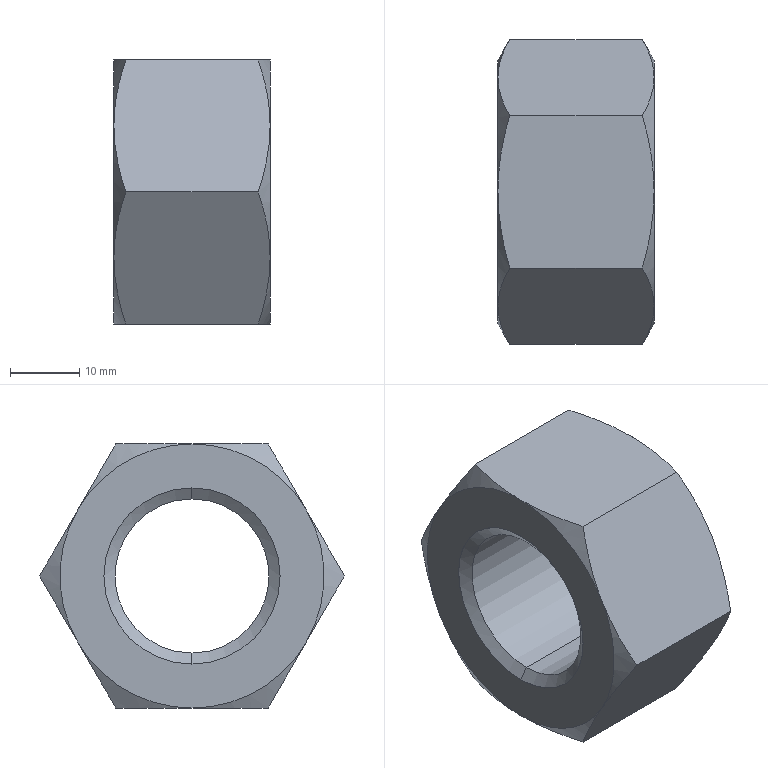Component | SolidWorks | hex thin nut chamfered gradeab_iso-1 | 1 solid | 28 faces | box 22.53 x 43.99 x 38.1 mm | volume 19330 mm3 | cone 16 | plane 8 | cylinder 4 | commonest cylinder face diameters 25.4 x2 22.225 x2
STEP:
#1=CARTESIAN_POINT('',(1.476,2.362,-4.831));
#2=VERTEX_POINT('',#1);
#3=CARTESIAN_POINT('',(1.476,2.362,-3.831));
#4=VERTEX_POINT('',#3);
#5=CARTESIAN_POINT('',(1.476,2.362,-4.331));
#6=DIRECTION('',(-1.,0.,0.));
#7=DIRECTION('',(0.,0.,-1.));
#8=AXIS2_PLACEMENT_3D('',#5,#6,#7);
#9=CIRCLE('',#8,0.5);
#10=EDGE_CURVE('',#2,#4,#9,.T.);
#11=ORIENTED_EDGE('',*,*,#10,.T.);
#12=CARTESIAN_POINT('',(1.477,2.362,-3.831));
#13=VERTEX_POINT('',#12);
#14=CARTESIAN_POINT('',(1.378,2.362,-3.831));
#15=DIRECTION('',(1.,0.,0.));
#16=VECTOR('',#15,39.37);
#17=LINE('',#14,#16);
#18=EDGE_CURVE('',#4,#13,#17,.T.);
#19=ORIENTED_EDGE('',*,*,#18,.T.);
#20=CARTESIAN_POINT('',(1.477,2.362,-4.831));
#21=VERTEX_POINT('',#20);
#22=CARTESIAN_POINT('',(1.477,2.362,-4.331));
#23=DIRECTION('',(1.,0.,0.));
#24=DIRECTION('',(0.,0.,-1.));
#25=AXIS2_PLACEMENT_3D('',#22,#23,#24);
#26=CIRCLE('',#25,0.5);
#27=EDGE_CURVE('',#13,#21,#26,.T.);
#28=ORIENTED_EDGE('',*,*,#27,.T.);
#29=CARTESIAN_POINT('',(1.378,2.362,-4.831));
#30=DIRECTION('',(1.,0.,0.));
#31=VECTOR('',#30,39.37);
#32=LINE('',#29,#31);
#33=EDGE_CURVE('',#2,#21,#32,.T.);
#34=ORIENTED_EDGE('',*,*,#33,.F.);
#35=EDGE_LOOP('',(#11,#19,#28,#34));
#36=FACE_OUTER_BOUND('',#35,.T.);
#37=CARTESIAN_POINT('',(1.378,2.362,-4.331));
#38=DIRECTION('',(1.,0.,0.));
#39=DIRECTION('',(0.,0.,-1.));
#40=AXIS2_PLACEMENT_3D('',#37,#38,#39);
#41=CYLINDRICAL_SURFACE('',#40,0.5);
#42=ADVANCED_FACE('',(#36),#41,.F.);
#43=CARTESIAN_POINT('',(1.521,2.362,-3.893));
#44=VERTEX_POINT('',#43);
#45=CARTESIAN_POINT('',(1.521,2.362,-4.768));
#46=VERTEX_POINT('',#45);
#47=CARTESIAN_POINT('',(1.521,2.362,-4.331));
#48=DIRECTION('',(1.,0.,0.));
#49=DIRECTION('',(0.,0.,1.));
#50=AXIS2_PLACEMENT_3D('',#47,#48,#49);
#51=CIRCLE('',#50,0.4375);
#52=EDGE_CURVE('',#44,#46,#51,.T.);
#53=ORIENTED_EDGE('',*,*,#52,.T.);
#54=CARTESIAN_POINT('',(1.477,2.362,-4.831));
#55=DIRECTION('',(-0.5736,0.,-0.8192));
#56=VECTOR('',#55,39.37);
#57=LINE('',#54,#56);
#58=EDGE_CURVE('',#46,#21,#57,.T.);
#59=ORIENTED_EDGE('',*,*,#58,.T.);
#60=ORIENTED_EDGE('',*,*,#27,.F.);
#61=CARTESIAN_POINT('',(1.477,2.362,-3.831));
#62=DIRECTION('',(-0.5736,0.,0.8192));
#63=VECTOR('',#62,39.37);
#64=LINE('',#61,#63);
#65=EDGE_CURVE('',#44,#13,#64,.T.);
#66=ORIENTED_EDGE('',*,*,#65,.F.);
#67=EDGE_LOOP('',(#53,#59,#60,#66));
#68=FACE_OUTER_BOUND('',#67,.T.);
#69=CARTESIAN_POINT('',(1.477,2.362,-4.331));
#70=DIRECTION('',(-1.,0.,0.));
#71=DIRECTION('',(0.,0.,1.));
#72=AXIS2_PLACEMENT_3D('',#69,#70,#71);
#73=CONICAL_SURFACE('',#72,0.5,0.9599);
#74=ADVANCED_FACE('',(#68),#73,.F.);
#75=CARTESIAN_POINT('',(2.32,2.362,-4.768));
#76=VERTEX_POINT('',#75);
#77=CARTESIAN_POINT('',(2.32,2.362,-3.893));
#78=VERTEX_POINT('',#77);
#79=CARTESIAN_POINT('',(2.32,2.362,-4.331));
#80=DIRECTION('',(-1.,0.,0.));
#81=DIRECTION('',(0.,0.,-1.));
#82=AXIS2_PLACEMENT_3D('',#79,#80,#81);
#83=CIRCLE('',#82,0.4375);
#84=EDGE_CURVE('',#76,#78,#83,.T.);
#85=ORIENTED_EDGE('',*,*,#84,.T.);
#86=CARTESIAN_POINT('',(2.363,2.362,-3.831));
#87=VERTEX_POINT('',#86);
#88=CARTESIAN_POINT('',(2.315,2.362,-3.899));
#89=DIRECTION('',(0.5736,0.,0.8192));
#90=VECTOR('',#89,39.37);
#91=LINE('',#88,#90);
#92=EDGE_CURVE('',#78,#87,#91,.T.);
#93=ORIENTED_EDGE('',*,*,#92,.T.);
#94=CARTESIAN_POINT('',(2.363,2.362,-4.831));
#95=VERTEX_POINT('',#94);
#96=CARTESIAN_POINT('',(2.363,2.362,-4.331));
#97=DIRECTION('',(1.,0.,0.));
#98=DIRECTION('',(0.,0.,-1.));
#99=AXIS2_PLACEMENT_3D('',#96,#97,#98);
#100=CIRCLE('',#99,0.5);
#101=EDGE_CURVE('',#87,#95,#100,.T.);
#102=ORIENTED_EDGE('',*,*,#101,.T.);
#103=CARTESIAN_POINT('',(2.315,2.362,-4.762));
#104=DIRECTION('',(0.5736,0.,-0.8192));
#105=VECTOR('',#104,39.37);
#106=LINE('',#103,#105);
#107=EDGE_CURVE('',#76,#95,#106,.T.);
#108=ORIENTED_EDGE('',*,*,#107,.F.);
#109=EDGE_LOOP('',(#85,#93,#102,#108));
#110=FACE_OUTER_BOUND('',#109,.T.);
#111=CARTESIAN_POINT('',(2.315,2.362,-4.331));
#112=DIRECTION('',(1.,0.,0.));
#113=DIRECTION('',(0.,0.,-1.));
#114=AXIS2_PLACEMENT_3D('',#111,#112,#113);
#115=CONICAL_SURFACE('',#114,0.4312,0.9599);
#116=ADVANCED_FACE('',(#110),#115,.F.);
#117=ORIENTED_EDGE('',*,*,#52,.F.);
#118=CARTESIAN_POINT('',(1.476,2.362,-3.893));
#119=DIRECTION('',(1.,0.,0.));
#120=VECTOR('',#119,39.37);
#121=LINE('',#118,#120);
#122=EDGE_CURVE('',#44,#78,#121,.T.);
#123=ORIENTED_EDGE('',*,*,#122,.T.);
#124=ORIENTED_EDGE('',*,*,#84,.F.);
#125=CARTESIAN_POINT('',(1.476,2.362,-4.768));
#126=DIRECTION('',(1.,0.,0.));
#127=VECTOR('',#126,39.37);
#128=LINE('',#125,#127);
#129=EDGE_CURVE('',#46,#76,#128,.T.);
#130=ORIENTED_EDGE('',*,*,#129,.F.);
#131=EDGE_LOOP('',(#117,#123,#124,#130));
#132=FACE_OUTER_BOUND('',#131,.T.);
#133=CARTESIAN_POINT('',(1.476,2.362,-4.331));
#134=DIRECTION('',(1.,0.,0.));
#135=DIRECTION('',(0.,0.,-1.));
#136=AXIS2_PLACEMENT_3D('',#133,#134,#135);
#137=CYLINDRICAL_SURFACE('',#136,0.4375);
#138=ADVANCED_FACE('',(#132),#137,.F.);
#139=ORIENTED_EDGE('',*,*,#122,.F.);
#140=CARTESIAN_POINT('',(1.521,2.362,-4.331));
#141=DIRECTION('',(1.,0.,0.));
#142=DIRECTION('',(0.,0.,1.));
#143=AXIS2_PLACEMENT_3D('',#140,#141,#142);
#144=CIRCLE('',#143,0.4375);
#145=EDGE_CURVE('',#46,#44,#144,.T.);
#146=ORIENTED_EDGE('',*,*,#145,.F.);
#147=ORIENTED_EDGE('',*,*,#129,.T.);
#148=CARTESIAN_POINT('',(2.32,2.362,-4.331));
#149=DIRECTION('',(-1.,0.,0.));
#150=DIRECTION('',(0.,0.,-1.));
#151=AXIS2_PLACEMENT_3D('',#148,#149,#150);
#152=CIRCLE('',#151,0.4375);
#153=EDGE_CURVE('',#78,#76,#152,.T.);
#154=ORIENTED_EDGE('',*,*,#153,.F.);
#155=EDGE_LOOP('',(#139,#146,#147,#154));
#156=FACE_OUTER_BOUND('',#155,.T.);
#157=CARTESIAN_POINT('',(1.476,2.362,-4.331));
#158=DIRECTION('',(1.,0.,0.));
#159=DIRECTION('',(0.,0.,-1.));
#160=AXIS2_PLACEMENT_3D('',#157,#158,#159);
#161=CYLINDRICAL_SURFACE('',#160,0.4375);
#162=ADVANCED_FACE('',(#156),#161,.F.);
#163=CARTESIAN_POINT('',(1.543,2.795,-3.581));
#164=VERTEX_POINT('',#163);
#165=CARTESIAN_POINT('',(2.296,2.795,-3.581));
#166=VERTEX_POINT('',#165);
#167=CARTESIAN_POINT('',(1.476,2.795,-3.581));
#168=DIRECTION('',(1.,0.,0.));
#169=VECTOR('',#168,39.37);
#170=LINE('',#167,#169);
#171=EDGE_CURVE('',#164,#166,#170,.T.);
#172=ORIENTED_EDGE('',*,*,#171,.T.);
#173=CARTESIAN_POINT('',(2.363,3.012,-3.956));
#174=VERTEX_POINT('',#173);
#175=CARTESIAN_POINT('',(2.296,2.795,-3.581));
#176=CARTESIAN_POINT('',(2.317,2.831,-3.642));
#177=CARTESIAN_POINT('',(2.334,2.866,-3.704));
#178=CARTESIAN_POINT('',(2.357,2.938,-3.829));
#179=CARTESIAN_POINT('',(2.363,2.975,-3.892));
#180=CARTESIAN_POINT('',(2.363,3.012,-3.956));
#181=B_SPLINE_CURVE_WITH_KNOTS('',3,(#175,#176,#177,#178,#179,#180),.UNSPECIFIED.,.F.,.F.,(4,2,4),(0.00000024,0.005565,0.01113),.UNSPECIFIED.);
#182=EDGE_CURVE('',#166,#174,#181,.T.);
#183=ORIENTED_EDGE('',*,*,#182,.T.);
#184=CARTESIAN_POINT('',(2.296,3.228,-4.331));
#185=VERTEX_POINT('',#184);
#186=CARTESIAN_POINT('',(2.363,3.012,-3.956));
#187=CARTESIAN_POINT('',(2.363,3.021,-3.972));
#188=CARTESIAN_POINT('',(2.363,3.03,-3.988));
#189=CARTESIAN_POINT('',(2.361,3.049,-4.019));
#190=CARTESIAN_POINT('',(2.36,3.058,-4.035));
#191=CARTESIAN_POINT('',(2.356,3.085,-4.083));
#192=CARTESIAN_POINT('',(2.351,3.103,-4.114));
#193=CARTESIAN_POINT('',(2.334,3.157,-4.208));
#194=CARTESIAN_POINT('',(2.317,3.193,-4.27));
#195=CARTESIAN_POINT('',(2.296,3.228,-4.331));
#196=B_SPLINE_CURVE_WITH_KNOTS('',3,(#186,#187,#188,#189,#190,#191,#192,#193,#194,#195),.UNSPECIFIED.,.F.,.F.,(4,2,2,2,4),(0.01113,0.01251,0.0139,0.01667,0.02222),.UNSPECIFIED.);
#197=EDGE_CURVE('',#174,#185,#196,.T.);
#198=ORIENTED_EDGE('',*,*,#197,.T.);
#199=CARTESIAN_POINT('',(1.543,3.228,-4.331));
#200=VERTEX_POINT('',#199);
#201=CARTESIAN_POINT('',(1.476,3.228,-4.331));
#202=DIRECTION('',(1.,0.,0.));
#203=VECTOR('',#202,39.37);
#204=LINE('',#201,#203);
#205=EDGE_CURVE('',#200,#185,#204,.T.);
#206=ORIENTED_EDGE('',*,*,#205,.F.);
#207=CARTESIAN_POINT('',(1.476,3.012,-3.956));
#208=VERTEX_POINT('',#207);
#209=CARTESIAN_POINT('',(1.476,3.012,-3.956));
#210=CARTESIAN_POINT('',(1.476,3.021,-3.972));
#211=CARTESIAN_POINT('',(1.477,3.03,-3.988));
#212=CARTESIAN_POINT('',(1.478,3.049,-4.019));
#213=CARTESIAN_POINT('',(1.479,3.058,-4.035));
#214=CARTESIAN_POINT('',(1.484,3.085,-4.083));
#215=CARTESIAN_POINT('',(1.489,3.103,-4.114));
#216=CARTESIAN_POINT('',(1.506,3.157,-4.208));
#217=CARTESIAN_POINT('',(1.523,3.193,-4.27));
#218=CARTESIAN_POINT('',(1.543,3.228,-4.331));
#219=B_SPLINE_CURVE_WITH_KNOTS('',3,(#209,#210,#211,#212,#213,#214,#215,#216,#217,#218),.UNSPECIFIED.,.F.,.F.,(4,2,2,2,4),(0.01113,0.01251,0.0139,0.01667,0.02222),.UNSPECIFIED.);
#220=EDGE_CURVE('',#208,#200,#219,.T.);
#221=ORIENTED_EDGE('',*,*,#220,.F.);
#222=CARTESIAN_POINT('',(1.543,2.795,-3.581));
#223=CARTESIAN_POINT('',(1.523,2.831,-3.642));
#224=CARTESIAN_POINT('',(1.506,2.866,-3.704));
#225=CARTESIAN_POINT('',(1.483,2.938,-3.829));
#226=CARTESIAN_POINT('',(1.476,2.975,-3.892));
#227=CARTESIAN_POINT('',(1.476,3.012,-3.956));
#228=B_SPLINE_CURVE_WITH_KNOTS('',3,(#222,#223,#224,#225,#226,#227),.UNSPECIFIED.,.F.,.F.,(4,2,4),(0.00000024,0.005565,0.01113),.UNSPECIFIED.);
#229=EDGE_CURVE('',#164,#208,#228,.T.);
#230=ORIENTED_EDGE('',*,*,#229,.F.);
#231=EDGE_LOOP('',(#172,#183,#198,#206,#221,#230));
#232=FACE_OUTER_BOUND('',#231,.T.);
#233=CARTESIAN_POINT('',(1.476,3.228,-4.331));
#234=DIRECTION('',(0.,0.866,0.5));
#235=DIRECTION('',(0.,-0.5,0.866));
#236=AXIS2_PLACEMENT_3D('',#233,#234,#235);
#237=PLANE('',#236);
#238=ADVANCED_FACE('',(#232),#237,.T.);
#239=ORIENTED_EDGE('',*,*,#205,.T.);
#240=CARTESIAN_POINT('',(2.363,3.012,-4.706));
#241=VERTEX_POINT('',#240);
#242=CARTESIAN_POINT('',(2.296,3.228,-4.331));
#243=CARTESIAN_POINT('',(2.317,3.193,-4.392));
#244=CARTESIAN_POINT('',(2.334,3.157,-4.454));
#245=CARTESIAN_POINT('',(2.357,3.085,-4.579));
#246=CARTESIAN_POINT('',(2.363,3.049,-4.642));
#247=CARTESIAN_POINT('',(2.363,3.012,-4.706));
#248=B_SPLINE_CURVE_WITH_KNOTS('',3,(#242,#243,#244,#245,#246,#247),.UNSPECIFIED.,.F.,.F.,(4,2,4),(0.00000024,0.005565,0.01113),.UNSPECIFIED.);
#249=EDGE_CURVE('',#185,#241,#248,.T.);
#250=ORIENTED_EDGE('',*,*,#249,.T.);
#251=CARTESIAN_POINT('',(2.296,2.795,-5.081));
#252=VERTEX_POINT('',#251);
#253=CARTESIAN_POINT('',(2.363,3.012,-4.706));
#254=CARTESIAN_POINT('',(2.363,3.003,-4.722));
#255=CARTESIAN_POINT('',(2.363,2.993,-4.738));
#256=CARTESIAN_POINT('',(2.361,2.975,-4.769));
#257=CARTESIAN_POINT('',(2.36,2.966,-4.785));
#258=CARTESIAN_POINT('',(2.356,2.938,-4.833));
#259=CARTESIAN_POINT('',(2.351,2.92,-4.864));
#260=CARTESIAN_POINT('',(2.334,2.866,-4.958));
#261=CARTESIAN_POINT('',(2.317,2.831,-5.02));
#262=CARTESIAN_POINT('',(2.296,2.795,-5.081));
#263=B_SPLINE_CURVE_WITH_KNOTS('',3,(#253,#254,#255,#256,#257,#258,#259,#260,#261,#262),.UNSPECIFIED.,.F.,.F.,(4,2,2,2,4),(0.01113,0.01251,0.0139,0.01667,0.02222),.UNSPECIFIED.);
#264=EDGE_CURVE('',#241,#252,#263,.T.);
#265=ORIENTED_EDGE('',*,*,#264,.T.);
#266=CARTESIAN_POINT('',(1.543,2.795,-5.081));
#267=VERTEX_POINT('',#266);
#268=CARTESIAN_POINT('',(1.476,2.795,-5.081));
#269=DIRECTION('',(1.,0.,0.));
#270=VECTOR('',#269,39.37);
#271=LINE('',#268,#270);
#272=EDGE_CURVE('',#267,#252,#271,.T.);
#273=ORIENTED_EDGE('',*,*,#272,.F.);
#274=CARTESIAN_POINT('',(1.476,3.012,-4.706));
#275=VERTEX_POINT('',#274);
#276=CARTESIAN_POINT('',(1.476,3.012,-4.706));
#277=CARTESIAN_POINT('',(1.476,3.003,-4.722));
#278=CARTESIAN_POINT('',(1.477,2.993,-4.738));
#279=CARTESIAN_POINT('',(1.478,2.975,-4.769));
#280=CARTESIAN_POINT('',(1.479,2.966,-4.785));
#281=CARTESIAN_POINT('',(1.484,2.938,-4.833));
#282=CARTESIAN_POINT('',(1.489,2.92,-4.864));
#283=CARTESIAN_POINT('',(1.506,2.866,-4.958));
#284=CARTESIAN_POINT('',(1.523,2.831,-5.02));
#285=CARTESIAN_POINT('',(1.543,2.795,-5.081));
#286=B_SPLINE_CURVE_WITH_KNOTS('',3,(#276,#277,#278,#279,#280,#281,#282,#283,#284,#285),.UNSPECIFIED.,.F.,.F.,(4,2,2,2,4),(0.01113,0.01251,0.0139,0.01667,0.02222),.UNSPECIFIED.);
#287=EDGE_CURVE('',#275,#267,#286,.T.);
#288=ORIENTED_EDGE('',*,*,#287,.F.);
#289=CARTESIAN_POINT('',(1.543,3.228,-4.331));
#290=CARTESIAN_POINT('',(1.523,3.193,-4.392));
#291=CARTESIAN_POINT('',(1.506,3.157,-4.454));
#292=CARTESIAN_POINT('',(1.483,3.085,-4.579));
#293=CARTESIAN_POINT('',(1.476,3.049,-4.642));
#294=CARTESIAN_POINT('',(1.476,3.012,-4.706));
#295=B_SPLINE_CURVE_WITH_KNOTS('',3,(#289,#290,#291,#292,#293,#294),.UNSPECIFIED.,.F.,.F.,(4,2,4),(0.00000024,0.005565,0.01113),.UNSPECIFIED.);
#296=EDGE_CURVE('',#200,#275,#295,.T.);
#297=ORIENTED_EDGE('',*,*,#296,.F.);
#298=EDGE_LOOP('',(#239,#250,#265,#273,#288,#297));
#299=FACE_OUTER_BOUND('',#298,.T.);
#300=CARTESIAN_POINT('',(1.476,2.795,-5.081));
#301=DIRECTION('',(0.,0.866,-0.5));
#302=DIRECTION('',(0.,0.5,0.866));
#303=AXIS2_PLACEMENT_3D('',#300,#301,#302);
#304=PLANE('',#303);
#305=ADVANCED_FACE('',(#299),#304,.T.);
#306=CARTESIAN_POINT('',(2.296,1.929,-5.081));
#307=VERTEX_POINT('',#306);
#308=CARTESIAN_POINT('',(2.363,2.362,-5.081));
#309=VERTEX_POINT('',#308);
#310=CARTESIAN_POINT('',(2.296,1.929,-5.081));
#311=CARTESIAN_POINT('',(2.307,1.964,-5.081));
#312=CARTESIAN_POINT('',(2.316,2.,-5.081));
#313=CARTESIAN_POINT('',(2.332,2.072,-5.081));
#314=CARTESIAN_POINT('',(2.34,2.108,-5.081));
#315=CARTESIAN_POINT('',(2.357,2.216,-5.081));
#316=CARTESIAN_POINT('',(2.363,2.289,-5.081));
#317=CARTESIAN_POINT('',(2.363,2.362,-5.081));
#318=B_SPLINE_CURVE_WITH_KNOTS('',3,(#310,#311,#312,#313,#314,#315,#316,#317),.UNSPECIFIED.,.F.,.F.,(4,2,2,4),(0.01962,0.0224,0.02519,0.03075),.UNSPECIFIED.);
#319=EDGE_CURVE('',#307,#309,#318,.T.);
#320=ORIENTED_EDGE('',*,*,#319,.F.);
#321=CARTESIAN_POINT('',(1.543,1.929,-5.081));
#322=VERTEX_POINT('',#321);
#323=CARTESIAN_POINT('',(1.476,1.929,-5.081));
#324=DIRECTION('',(1.,0.,0.));
#325=VECTOR('',#324,39.37);
#326=LINE('',#323,#325);
#327=EDGE_CURVE('',#322,#307,#326,.T.);
#328=ORIENTED_EDGE('',*,*,#327,.F.);
#329=CARTESIAN_POINT('',(1.476,2.362,-5.081));
#330=VERTEX_POINT('',#329);
#331=CARTESIAN_POINT('',(1.543,1.929,-5.081));
#332=CARTESIAN_POINT('',(1.533,1.964,-5.081));
#333=CARTESIAN_POINT('',(1.524,2.,-5.081));
#334=CARTESIAN_POINT('',(1.507,2.072,-5.081));
#335=CARTESIAN_POINT('',(1.5,2.108,-5.081));
#336=CARTESIAN_POINT('',(1.483,2.216,-5.081));
#337=CARTESIAN_POINT('',(1.476,2.289,-5.081));
#338=CARTESIAN_POINT('',(1.476,2.362,-5.081));
#339=B_SPLINE_CURVE_WITH_KNOTS('',3,(#331,#332,#333,#334,#335,#336,#337,#338),.UNSPECIFIED.,.F.,.F.,(4,2,2,4),(0.01962,0.0224,0.02519,0.03075),.UNSPECIFIED.);
#340=EDGE_CURVE('',#322,#330,#339,.T.);
#341=ORIENTED_EDGE('',*,*,#340,.T.);
#342=CARTESIAN_POINT('',(1.476,2.362,-5.081));
#343=CARTESIAN_POINT('',(1.476,2.399,-5.081));
#344=CARTESIAN_POINT('',(1.478,2.436,-5.081));
#345=CARTESIAN_POINT('',(1.484,2.509,-5.081));
#346=CARTESIAN_POINT('',(1.489,2.546,-5.081));
#347=CARTESIAN_POINT('',(1.506,2.654,-5.081));
#348=CARTESIAN_POINT('',(1.523,2.725,-5.081));
#349=CARTESIAN_POINT('',(1.543,2.795,-5.081));
#350=B_SPLINE_CURVE_WITH_KNOTS('',3,(#342,#343,#344,#345,#346,#347,#348,#349),.UNSPECIFIED.,.F.,.F.,(4,2,2,4),(0.03075,0.03353,0.03632,0.04188),.UNSPECIFIED.);
#351=EDGE_CURVE('',#330,#267,#350,.T.);
#352=ORIENTED_EDGE('',*,*,#351,.T.);
#353=ORIENTED_EDGE('',*,*,#272,.T.);
#354=CARTESIAN_POINT('',(2.363,2.362,-5.081));
#355=CARTESIAN_POINT('',(2.363,2.399,-5.081));
#356=CARTESIAN_POINT('',(2.362,2.436,-5.081));
#357=CARTESIAN_POINT('',(2.356,2.509,-5.081));
#358=CARTESIAN_POINT('',(2.351,2.546,-5.081));
#359=CARTESIAN_POINT('',(2.333,2.654,-5.081));
#360=CARTESIAN_POINT('',(2.317,2.725,-5.081));
#361=CARTESIAN_POINT('',(2.296,2.795,-5.081));
#362=B_SPLINE_CURVE_WITH_KNOTS('',3,(#354,#355,#356,#357,#358,#359,#360,#361),.UNSPECIFIED.,.F.,.F.,(4,2,2,4),(0.03075,0.03353,0.03632,0.04188),.UNSPECIFIED.);
#363=EDGE_CURVE('',#309,#252,#362,.T.);
#364=ORIENTED_EDGE('',*,*,#363,.F.);
#365=EDGE_LOOP('',(#320,#328,#341,#352,#353,#364));
#366=FACE_OUTER_BOUND('',#365,.T.);
#367=CARTESIAN_POINT('',(1.476,2.795,-5.081));
#368=DIRECTION('',(0.,0.,1.));
#369=DIRECTION('',(1.,0.,0.));
#370=AXIS2_PLACEMENT_3D('',#367,#368,#369);
#371=PLANE('',#370);
#372=ADVANCED_FACE('',(#366),#371,.F.);
#373=ORIENTED_EDGE('',*,*,#327,.T.);
#374=CARTESIAN_POINT('',(2.363,1.713,-4.706));
#375=VERTEX_POINT('',#374);
#376=CARTESIAN_POINT('',(2.296,1.929,-5.081));
#377=CARTESIAN_POINT('',(2.317,1.894,-5.019));
#378=CARTESIAN_POINT('',(2.334,1.858,-4.958));
#379=CARTESIAN_POINT('',(2.357,1.786,-4.833));
#380=CARTESIAN_POINT('',(2.363,1.75,-4.77));
#381=CARTESIAN_POINT('',(2.363,1.713,-4.706));
#382=B_SPLINE_CURVE_WITH_KNOTS('',3,(#376,#377,#378,#379,#380,#381),.UNSPECIFIED.,.F.,.F.,(4,2,4),(0.00000024,0.005565,0.01113),.UNSPECIFIED.);
#383=EDGE_CURVE('',#307,#375,#382,.T.);
#384=ORIENTED_EDGE('',*,*,#383,.T.);
#385=CARTESIAN_POINT('',(2.296,1.496,-4.331));
#386=VERTEX_POINT('',#385);
#387=CARTESIAN_POINT('',(2.363,1.713,-4.706));
#388=CARTESIAN_POINT('',(2.363,1.703,-4.69));
#389=CARTESIAN_POINT('',(2.363,1.694,-4.674));
#390=CARTESIAN_POINT('',(2.361,1.676,-4.642));
#391=CARTESIAN_POINT('',(2.36,1.667,-4.626));
#392=CARTESIAN_POINT('',(2.356,1.639,-4.579));
#393=CARTESIAN_POINT('',(2.351,1.621,-4.547));
#394=CARTESIAN_POINT('',(2.334,1.567,-4.454));
#395=CARTESIAN_POINT('',(2.317,1.532,-4.392));
#396=CARTESIAN_POINT('',(2.296,1.496,-4.331));
#397=B_SPLINE_CURVE_WITH_KNOTS('',3,(#387,#388,#389,#390,#391,#392,#393,#394,#395,#396),.UNSPECIFIED.,.F.,.F.,(4,2,2,2,4),(0.01113,0.01251,0.0139,0.01667,0.02222),.UNSPECIFIED.);
#398=EDGE_CURVE('',#375,#386,#397,.T.);
#399=ORIENTED_EDGE('',*,*,#398,.T.);
#400=CARTESIAN_POINT('',(1.543,1.496,-4.331));
#401=VERTEX_POINT('',#400);
#402=CARTESIAN_POINT('',(1.476,1.496,-4.331));
#403=DIRECTION('',(1.,0.,0.));
#404=VECTOR('',#403,39.37);
#405=LINE('',#402,#404);
#406=EDGE_CURVE('',#401,#386,#405,.T.);
#407=ORIENTED_EDGE('',*,*,#406,.F.);
#408=CARTESIAN_POINT('',(1.476,1.713,-4.706));
#409=VERTEX_POINT('',#408);
#410=CARTESIAN_POINT('',(1.476,1.713,-4.706));
#411=CARTESIAN_POINT('',(1.476,1.703,-4.69));
#412=CARTESIAN_POINT('',(1.477,1.694,-4.674));
#413=CARTESIAN_POINT('',(1.478,1.676,-4.642));
#414=CARTESIAN_POINT('',(1.479,1.667,-4.626));
#415=CARTESIAN_POINT('',(1.484,1.639,-4.579));
#416=CARTESIAN_POINT('',(1.489,1.621,-4.547));
#417=CARTESIAN_POINT('',(1.506,1.567,-4.454));
#418=CARTESIAN_POINT('',(1.523,1.532,-4.392));
#419=CARTESIAN_POINT('',(1.543,1.496,-4.331));
#420=B_SPLINE_CURVE_WITH_KNOTS('',3,(#410,#411,#412,#413,#414,#415,#416,#417,#418,#419),.UNSPECIFIED.,.F.,.F.,(4,2,2,2,4),(0.01113,0.01251,0.0139,0.01667,0.02222),.UNSPECIFIED.);
#421=EDGE_CURVE('',#409,#401,#420,.T.);
#422=ORIENTED_EDGE('',*,*,#421,.F.);
#423=CARTESIAN_POINT('',(1.543,1.929,-5.081));
#424=CARTESIAN_POINT('',(1.523,1.894,-5.019));
#425=CARTESIAN_POINT('',(1.506,1.858,-4.958));
#426=CARTESIAN_POINT('',(1.483,1.786,-4.833));
#427=CARTESIAN_POINT('',(1.476,1.75,-4.77));
#428=CARTESIAN_POINT('',(1.476,1.713,-4.706));
#429=B_SPLINE_CURVE_WITH_KNOTS('',3,(#423,#424,#425,#426,#427,#428),.UNSPECIFIED.,.F.,.F.,(4,2,4),(0.00000024,0.005565,0.01113),.UNSPECIFIED.);
#430=EDGE_CURVE('',#322,#409,#429,.T.);
#431=ORIENTED_EDGE('',*,*,#430,.F.);
#432=EDGE_LOOP('',(#373,#384,#399,#407,#422,#431));
#433=FACE_OUTER_BOUND('',#432,.T.);
#434=CARTESIAN_POINT('',(1.476,1.496,-4.331));
#435=DIRECTION('',(0.,-0.866,-0.5));
#436=DIRECTION('',(0.,0.5,-0.866));
#437=AXIS2_PLACEMENT_3D('',#434,#435,#436);
#438=PLANE('',#437);
#439=ADVANCED_FACE('',(#433),#438,.T.);
#440=ORIENTED_EDGE('',*,*,#406,.T.);
#441=CARTESIAN_POINT('',(2.363,1.713,-3.956));
#442=VERTEX_POINT('',#441);
#443=CARTESIAN_POINT('',(2.296,1.496,-4.331));
#444=CARTESIAN_POINT('',(2.317,1.532,-4.269));
#445=CARTESIAN_POINT('',(2.334,1.567,-4.208));
#446=CARTESIAN_POINT('',(2.357,1.639,-4.083));
#447=CARTESIAN_POINT('',(2.363,1.676,-4.02));
#448=CARTESIAN_POINT('',(2.363,1.713,-3.956));
#449=B_SPLINE_CURVE_WITH_KNOTS('',3,(#443,#444,#445,#446,#447,#448),.UNSPECIFIED.,.F.,.F.,(4,2,4),(0.00000024,0.005565,0.01113),.UNSPECIFIED.);
#450=EDGE_CURVE('',#386,#442,#449,.T.);
#451=ORIENTED_EDGE('',*,*,#450,.T.);
#452=CARTESIAN_POINT('',(2.296,1.929,-3.581));
#453=VERTEX_POINT('',#452);
#454=CARTESIAN_POINT('',(2.363,1.713,-3.956));
#455=CARTESIAN_POINT('',(2.363,1.722,-3.94));
#456=CARTESIAN_POINT('',(2.363,1.731,-3.924));
#457=CARTESIAN_POINT('',(2.361,1.749,-3.892));
#458=CARTESIAN_POINT('',(2.36,1.759,-3.876));
#459=CARTESIAN_POINT('',(2.356,1.786,-3.829));
#460=CARTESIAN_POINT('',(2.351,1.804,-3.797));
#461=CARTESIAN_POINT('',(2.334,1.858,-3.704));
#462=CARTESIAN_POINT('',(2.317,1.894,-3.642));
#463=CARTESIAN_POINT('',(2.296,1.929,-3.581));
#464=B_SPLINE_CURVE_WITH_KNOTS('',3,(#454,#455,#456,#457,#458,#459,#460,#461,#462,#463),.UNSPECIFIED.,.F.,.F.,(4,2,2,2,4),(0.01113,0.01251,0.0139,0.01667,0.02222),.UNSPECIFIED.);
#465=EDGE_CURVE('',#442,#453,#464,.T.);
#466=ORIENTED_EDGE('',*,*,#465,.T.);
#467=CARTESIAN_POINT('',(1.543,1.929,-3.581));
#468=VERTEX_POINT('',#467);
#469=CARTESIAN_POINT('',(1.476,1.929,-3.581));
#470=DIRECTION('',(1.,0.,0.));
#471=VECTOR('',#470,39.37);
#472=LINE('',#469,#471);
#473=EDGE_CURVE('',#468,#453,#472,.T.);
#474=ORIENTED_EDGE('',*,*,#473,.F.);
#475=CARTESIAN_POINT('',(1.476,1.713,-3.956));
#476=VERTEX_POINT('',#475);
#477=CARTESIAN_POINT('',(1.476,1.713,-3.956));
#478=CARTESIAN_POINT('',(1.476,1.722,-3.94));
#479=CARTESIAN_POINT('',(1.477,1.731,-3.924));
#480=CARTESIAN_POINT('',(1.478,1.749,-3.892));
#481=CARTESIAN_POINT('',(1.479,1.759,-3.876));
#482=CARTESIAN_POINT('',(1.484,1.786,-3.829));
#483=CARTESIAN_POINT('',(1.489,1.804,-3.797));
#484=CARTESIAN_POINT('',(1.506,1.858,-3.704));
#485=CARTESIAN_POINT('',(1.523,1.894,-3.642));
#486=CARTESIAN_POINT('',(1.543,1.929,-3.581));
#487=B_SPLINE_CURVE_WITH_KNOTS('',3,(#477,#478,#479,#480,#481,#482,#483,#484,#485,#486),.UNSPECIFIED.,.F.,.F.,(4,2,2,2,4),(0.01113,0.01251,0.0139,0.01667,0.02222),.UNSPECIFIED.);
#488=EDGE_CURVE('',#476,#468,#487,.T.);
#489=ORIENTED_EDGE('',*,*,#488,.F.);
#490=CARTESIAN_POINT('',(1.543,1.496,-4.331));
#491=CARTESIAN_POINT('',(1.523,1.532,-4.269));
#492=CARTESIAN_POINT('',(1.506,1.567,-4.208));
#493=CARTESIAN_POINT('',(1.483,1.639,-4.083));
#494=CARTESIAN_POINT('',(1.476,1.676,-4.02));
#495=CARTESIAN_POINT('',(1.476,1.713,-3.956));
#496=B_SPLINE_CURVE_WITH_KNOTS('',3,(#490,#491,#492,#493,#494,#495),.UNSPECIFIED.,.F.,.F.,(4,2,4),(0.00000024,0.005565,0.01113),.UNSPECIFIED.);
#497=EDGE_CURVE('',#401,#476,#496,.T.);
#498=ORIENTED_EDGE('',*,*,#497,.F.);
#499=EDGE_LOOP('',(#440,#451,#466,#474,#489,#498));
#500=FACE_OUTER_BOUND('',#499,.T.);
#501=CARTESIAN_POINT('',(1.476,1.929,-3.581));
#502=DIRECTION('',(0.,-0.866,0.5));
#503=DIRECTION('',(0.,-0.5,-0.866));
#504=AXIS2_PLACEMENT_3D('',#501,#502,#503);
#505=PLANE('',#504);
#506=ADVANCED_FACE('',(#500),#505,.T.);
#507=ORIENTED_EDGE('',*,*,#473,.T.);
#508=CARTESIAN_POINT('',(2.363,2.362,-3.581));
#509=VERTEX_POINT('',#508);
#510=CARTESIAN_POINT('',(2.296,1.929,-3.581));
#511=CARTESIAN_POINT('',(2.307,1.964,-3.581));
#512=CARTESIAN_POINT('',(2.316,2.,-3.581));
#513=CARTESIAN_POINT('',(2.332,2.072,-3.581));
#514=CARTESIAN_POINT('',(2.34,2.108,-3.581));
#515=CARTESIAN_POINT('',(2.357,2.216,-3.581));
#516=CARTESIAN_POINT('',(2.363,2.289,-3.581));
#517=CARTESIAN_POINT('',(2.363,2.362,-3.581));
#518=B_SPLINE_CURVE_WITH_KNOTS('',3,(#510,#511,#512,#513,#514,#515,#516,#517),.UNSPECIFIED.,.F.,.F.,(4,2,2,4),(0.01962,0.0224,0.02519,0.03075),.UNSPECIFIED.);
#519=EDGE_CURVE('',#453,#509,#518,.T.);
#520=ORIENTED_EDGE('',*,*,#519,.T.);
#521=CARTESIAN_POINT('',(2.363,2.362,-3.581));
#522=CARTESIAN_POINT('',(2.363,2.399,-3.581));
#523=CARTESIAN_POINT('',(2.362,2.436,-3.581));
#524=CARTESIAN_POINT('',(2.356,2.509,-3.581));
#525=CARTESIAN_POINT('',(2.351,2.546,-3.581));
#526=CARTESIAN_POINT('',(2.333,2.654,-3.581));
#527=CARTESIAN_POINT('',(2.317,2.725,-3.581));
#528=CARTESIAN_POINT('',(2.296,2.795,-3.581));
#529=B_SPLINE_CURVE_WITH_KNOTS('',3,(#521,#522,#523,#524,#525,#526,#527,#528),.UNSPECIFIED.,.F.,.F.,(4,2,2,4),(0.03075,0.03353,0.03632,0.04188),.UNSPECIFIED.);
#530=EDGE_CURVE('',#509,#166,#529,.T.);
#531=ORIENTED_EDGE('',*,*,#530,.T.);
#532=ORIENTED_EDGE('',*,*,#171,.F.);
#533=CARTESIAN_POINT('',(1.476,2.362,-3.581));
#534=VERTEX_POINT('',#533);
#535=CARTESIAN_POINT('',(1.476,2.362,-3.581));
#536=CARTESIAN_POINT('',(1.476,2.399,-3.581));
#537=CARTESIAN_POINT('',(1.478,2.436,-3.581));
#538=CARTESIAN_POINT('',(1.484,2.509,-3.581));
#539=CARTESIAN_POINT('',(1.489,2.546,-3.581));
#540=CARTESIAN_POINT('',(1.506,2.654,-3.581));
#541=CARTESIAN_POINT('',(1.523,2.725,-3.581));
#542=CARTESIAN_POINT('',(1.543,2.795,-3.581));
#543=B_SPLINE_CURVE_WITH_KNOTS('',3,(#535,#536,#537,#538,#539,#540,#541,#542),.UNSPECIFIED.,.F.,.F.,(4,2,2,4),(0.03075,0.03353,0.03632,0.04188),.UNSPECIFIED.);
#544=EDGE_CURVE('',#534,#164,#543,.T.);
#545=ORIENTED_EDGE('',*,*,#544,.F.);
#546=CARTESIAN_POINT('',(1.543,1.929,-3.581));
#547=CARTESIAN_POINT('',(1.533,1.964,-3.581));
#548=CARTESIAN_POINT('',(1.524,2.,-3.581));
#549=CARTESIAN_POINT('',(1.507,2.072,-3.581));
#550=CARTESIAN_POINT('',(1.5,2.108,-3.581));
#551=CARTESIAN_POINT('',(1.483,2.216,-3.581));
#552=CARTESIAN_POINT('',(1.476,2.289,-3.581));
#553=CARTESIAN_POINT('',(1.476,2.362,-3.581));
#554=B_SPLINE_CURVE_WITH_KNOTS('',3,(#546,#547,#548,#549,#550,#551,#552,#553),.UNSPECIFIED.,.F.,.F.,(4,2,2,4),(0.01962,0.0224,0.02519,0.03075),.UNSPECIFIED.);
#555=EDGE_CURVE('',#468,#534,#554,.T.);
#556=ORIENTED_EDGE('',*,*,#555,.F.);
#557=EDGE_LOOP('',(#507,#520,#531,#532,#545,#556));
#558=FACE_OUTER_BOUND('',#557,.T.);
#559=CARTESIAN_POINT('',(1.476,2.795,-3.581));
#560=DIRECTION('',(0.,0.,1.));
#561=DIRECTION('',(1.,0.,0.));
#562=AXIS2_PLACEMENT_3D('',#559,#560,#561);
#563=PLANE('',#562);
#564=ADVANCED_FACE('',(#558),#563,.T.);
#565=CARTESIAN_POINT('',(2.363,2.362,-4.331));
#566=DIRECTION('',(1.,0.,0.));
#567=DIRECTION('',(0.,0.,-1.));
#568=AXIS2_PLACEMENT_3D('',#565,#566,#567);
#569=CIRCLE('',#568,0.5);
#570=EDGE_CURVE('',#95,#87,#569,.T.);
#571=ORIENTED_EDGE('',*,*,#570,.F.);
#572=ORIENTED_EDGE('',*,*,#101,.F.);
#573=EDGE_LOOP('',(#571,#572));
#574=FACE_BOUND('',#573,.T.);
#575=CARTESIAN_POINT('',(2.363,2.362,-4.331));
#576=DIRECTION('',(1.,0.,0.));
#577=DIRECTION('',(0.,0.,-1.));
#578=AXIS2_PLACEMENT_3D('',#575,#576,#577);
#579=CIRCLE('',#578,0.75);
#580=EDGE_CURVE('',#375,#309,#579,.T.);
#581=ORIENTED_EDGE('',*,*,#580,.T.);
#582=CARTESIAN_POINT('',(2.363,2.362,-4.331));
#583=DIRECTION('',(1.,0.,0.));
#584=DIRECTION('',(0.,0.,-1.));
#585=AXIS2_PLACEMENT_3D('',#582,#583,#584);
#586=CIRCLE('',#585,0.75);
#587=EDGE_CURVE('',#309,#241,#586,.T.);
#588=ORIENTED_EDGE('',*,*,#587,.T.);
#589=CARTESIAN_POINT('',(2.363,2.362,-4.331));
#590=DIRECTION('',(1.,0.,0.));
#591=DIRECTION('',(0.,0.,-1.));
#592=AXIS2_PLACEMENT_3D('',#589,#590,#591);
#593=CIRCLE('',#592,0.75);
#594=EDGE_CURVE('',#241,#174,#593,.T.);
#595=ORIENTED_EDGE('',*,*,#594,.T.);
#596=CARTESIAN_POINT('',(2.363,2.362,-4.331));
#597=DIRECTION('',(1.,0.,0.));
#598=DIRECTION('',(0.,0.,-1.));
#599=AXIS2_PLACEMENT_3D('',#596,#597,#598);
#600=CIRCLE('',#599,0.75);
#601=EDGE_CURVE('',#174,#509,#600,.T.);
#602=ORIENTED_EDGE('',*,*,#601,.T.);
#603=CARTESIAN_POINT('',(2.363,2.362,-4.331));
#604=DIRECTION('',(1.,0.,0.));
#605=DIRECTION('',(0.,0.,-1.));
#606=AXIS2_PLACEMENT_3D('',#603,#604,#605);
#607=CIRCLE('',#606,0.75);
#608=EDGE_CURVE('',#509,#442,#607,.T.);
#609=ORIENTED_EDGE('',*,*,#608,.T.);
#610=CARTESIAN_POINT('',(2.363,2.362,-4.331));
#611=DIRECTION('',(1.,0.,0.));
#612=DIRECTION('',(0.,0.,-1.));
#613=AXIS2_PLACEMENT_3D('',#610,#611,#612);
#614=CIRCLE('',#613,0.75);
#615=EDGE_CURVE('',#442,#375,#614,.T.);
#616=ORIENTED_EDGE('',*,*,#615,.T.);
#617=EDGE_LOOP('',(#581,#588,#595,#602,#609,#616));
#618=FACE_OUTER_BOUND('',#617,.T.);
#619=CARTESIAN_POINT('',(2.363,2.362,-2.831));
#620=DIRECTION('',(1.,0.,0.));
#621=DIRECTION('',(0.,0.,-1.));
#622=AXIS2_PLACEMENT_3D('',#619,#620,#621);
#623=PLANE('',#622);
#624=ADVANCED_FACE('',(#574,#618),#623,.T.);
#625=ORIENTED_EDGE('',*,*,#10,.F.);
#626=CARTESIAN_POINT('',(1.476,2.362,-4.331));
#627=DIRECTION('',(-1.,0.,0.));
#628=DIRECTION('',(0.,0.,-1.));
#629=AXIS2_PLACEMENT_3D('',#626,#627,#628);
#630=CIRCLE('',#629,0.5);
#631=EDGE_CURVE('',#4,#2,#630,.T.);
#632=ORIENTED_EDGE('',*,*,#631,.F.);
#633=EDGE_LOOP('',(#625,#632));
#634=FACE_BOUND('',#633,.T.);
#635=CARTESIAN_POINT('',(1.476,2.362,-4.331));
#636=DIRECTION('',(1.,0.,0.));
#637=DIRECTION('',(0.,0.,-1.));
#638=AXIS2_PLACEMENT_3D('',#635,#636,#637);
#639=CIRCLE('',#638,0.75);
#640=EDGE_CURVE('',#330,#275,#639,.T.);
#641=ORIENTED_EDGE('',*,*,#640,.F.);
#642=CARTESIAN_POINT('',(1.476,2.362,-4.331));
#643=DIRECTION('',(-1.,0.,0.));
#644=DIRECTION('',(0.,0.,-1.));
#645=AXIS2_PLACEMENT_3D('',#642,#643,#644);
#646=CIRCLE('',#645,0.75);
#647=EDGE_CURVE('',#330,#409,#646,.T.);
#648=ORIENTED_EDGE('',*,*,#647,.T.);
#649=CARTESIAN_POINT('',(1.476,2.362,-4.331));
#650=DIRECTION('',(-1.,0.,0.));
#651=DIRECTION('',(0.,0.,-1.));
#652=AXIS2_PLACEMENT_3D('',#649,#650,#651);
#653=CIRCLE('',#652,0.75);
#654=EDGE_CURVE('',#409,#476,#653,.T.);
#655=ORIENTED_EDGE('',*,*,#654,.T.);
#656=CARTESIAN_POINT('',(1.476,2.362,-4.331));
#657=DIRECTION('',(-1.,0.,0.));
#658=DIRECTION('',(0.,0.,-1.));
#659=AXIS2_PLACEMENT_3D('',#656,#657,#658);
#660=CIRCLE('',#659,0.75);
#661=EDGE_CURVE('',#476,#534,#660,.T.);
#662=ORIENTED_EDGE('',*,*,#661,.T.);
#663=CARTESIAN_POINT('',(1.476,2.362,-4.331));
#664=DIRECTION('',(-1.,0.,0.));
#665=DIRECTION('',(0.,0.,-1.));
#666=AXIS2_PLACEMENT_3D('',#663,#664,#665);
#667=CIRCLE('',#666,0.75);
#668=EDGE_CURVE('',#534,#208,#667,.T.);
#669=ORIENTED_EDGE('',*,*,#668,.T.);
#670=CARTESIAN_POINT('',(1.476,2.362,-4.331));
#671=DIRECTION('',(-1.,0.,0.));
#672=DIRECTION('',(0.,-0.,-1.));
#673=AXIS2_PLACEMENT_3D('',#670,#671,#672);
#674=CIRCLE('',#673,0.75);
#675=EDGE_CURVE('',#208,#275,#674,.T.);
#676=ORIENTED_EDGE('',*,*,#675,.T.);
#677=EDGE_LOOP('',(#641,#648,#655,#662,#669,#676));
#678=FACE_OUTER_BOUND('',#677,.T.);
#679=CARTESIAN_POINT('',(1.476,2.362,-2.831));
#680=DIRECTION('',(1.,0.,0.));
#681=DIRECTION('',(0.,0.,-1.));
#682=AXIS2_PLACEMENT_3D('',#679,#680,#681);
#683=PLANE('',#682);
#684=ADVANCED_FACE('',(#634,#678),#683,.F.);
#685=ORIENTED_EDGE('',*,*,#287,.T.);
#686=ORIENTED_EDGE('',*,*,#351,.F.);
#687=ORIENTED_EDGE('',*,*,#640,.T.);
#688=EDGE_LOOP('',(#685,#686,#687));
#689=FACE_OUTER_BOUND('',#688,.T.);
#690=CARTESIAN_POINT('',(1.476,2.362,-4.331));
#691=DIRECTION('',(1.,0.,0.));
#692=DIRECTION('',(0.,0.,-1.));
#693=AXIS2_PLACEMENT_3D('',#690,#691,#692);
#694=CONICAL_SURFACE('',#693,0.75,1.047);
#695=ADVANCED_FACE('',(#689),#694,.T.);
#696=ORIENTED_EDGE('',*,*,#220,.T.);
#697=ORIENTED_EDGE('',*,*,#296,.T.);
#698=ORIENTED_EDGE('',*,*,#675,.F.);
#699=EDGE_LOOP('',(#696,#697,#698));
#700=FACE_OUTER_BOUND('',#699,.T.);
#701=CARTESIAN_POINT('',(1.476,2.362,-4.331));
#702=DIRECTION('',(1.,0.,0.));
#703=DIRECTION('',(0.,0.,-1.));
#704=AXIS2_PLACEMENT_3D('',#701,#702,#703);
#705=CONICAL_SURFACE('',#704,0.75,1.047);
#706=ADVANCED_FACE('',(#700),#705,.T.);
#707=ORIENTED_EDGE('',*,*,#229,.T.);
#708=ORIENTED_EDGE('',*,*,#668,.F.);
#709=ORIENTED_EDGE('',*,*,#544,.T.);
#710=EDGE_LOOP('',(#707,#708,#709));
#711=FACE_OUTER_BOUND('',#710,.T.);
#712=CARTESIAN_POINT('',(1.476,2.362,-4.331));
#713=DIRECTION('',(1.,0.,0.));
#714=DIRECTION('',(0.,0.,-1.));
#715=AXIS2_PLACEMENT_3D('',#712,#713,#714);
#716=CONICAL_SURFACE('',#715,0.75,1.047);
#717=ADVANCED_FACE('',(#711),#716,.T.);
#718=ORIENTED_EDGE('',*,*,#488,.T.);
#719=ORIENTED_EDGE('',*,*,#555,.T.);
#720=ORIENTED_EDGE('',*,*,#661,.F.);
#721=EDGE_LOOP('',(#718,#719,#720));
#722=FACE_OUTER_BOUND('',#721,.T.);
#723=CARTESIAN_POINT('',(1.476,2.362,-4.331));
#724=DIRECTION('',(1.,0.,0.));
#725=DIRECTION('',(0.,0.,-1.));
#726=AXIS2_PLACEMENT_3D('',#723,#724,#725);
#727=CONICAL_SURFACE('',#726,0.75,1.047);
#728=ADVANCED_FACE('',(#722),#727,.T.);
#729=ORIENTED_EDGE('',*,*,#421,.T.);
#730=ORIENTED_EDGE('',*,*,#497,.T.);
#731=ORIENTED_EDGE('',*,*,#654,.F.);
#732=EDGE_LOOP('',(#729,#730,#731));
#733=FACE_OUTER_BOUND('',#732,.T.);
#734=CARTESIAN_POINT('',(1.476,2.362,-4.331));
#735=DIRECTION('',(1.,0.,0.));
#736=DIRECTION('',(0.,0.,-1.));
#737=AXIS2_PLACEMENT_3D('',#734,#735,#736);
#738=CONICAL_SURFACE('',#737,0.75,1.047);
#739=ADVANCED_FACE('',(#733),#738,.T.);
#740=ORIENTED_EDGE('',*,*,#430,.T.);
#741=ORIENTED_EDGE('',*,*,#647,.F.);
#742=ORIENTED_EDGE('',*,*,#340,.F.);
#743=EDGE_LOOP('',(#740,#741,#742));
#744=FACE_OUTER_BOUND('',#743,.T.);
#745=CARTESIAN_POINT('',(1.476,2.362,-4.331));
#746=DIRECTION('',(1.,0.,0.));
#747=DIRECTION('',(0.,0.,-1.));
#748=AXIS2_PLACEMENT_3D('',#745,#746,#747);
#749=CONICAL_SURFACE('',#748,0.75,1.047);
#750=ADVANCED_FACE('',(#744),#749,.T.);
#751=ORIENTED_EDGE('',*,*,#319,.T.);
#752=ORIENTED_EDGE('',*,*,#580,.F.);
#753=ORIENTED_EDGE('',*,*,#383,.F.);
#754=EDGE_LOOP('',(#751,#752,#753));
#755=FACE_OUTER_BOUND('',#754,.T.);
#756=CARTESIAN_POINT('',(2.363,2.362,-4.331));
#757=DIRECTION('',(-1.,0.,0.));
#758=DIRECTION('',(0.,0.,1.));
#759=AXIS2_PLACEMENT_3D('',#756,#757,#758);
#760=CONICAL_SURFACE('',#759,0.75,1.047);
#761=ADVANCED_FACE('',(#755),#760,.T.);
#762=ORIENTED_EDGE('',*,*,#615,.F.);
#763=ORIENTED_EDGE('',*,*,#450,.F.);
#764=ORIENTED_EDGE('',*,*,#398,.F.);
#765=EDGE_LOOP('',(#762,#763,#764));
#766=FACE_OUTER_BOUND('',#765,.T.);
#767=CARTESIAN_POINT('',(2.363,2.362,-4.331));
#768=DIRECTION('',(-1.,0.,0.));
#769=DIRECTION('',(0.,0.,1.));
#770=AXIS2_PLACEMENT_3D('',#767,#768,#769);
#771=CONICAL_SURFACE('',#770,0.75,1.047);
#772=ADVANCED_FACE('',(#766),#771,.T.);
#773=ORIENTED_EDGE('',*,*,#608,.F.);
#774=ORIENTED_EDGE('',*,*,#519,.F.);
#775=ORIENTED_EDGE('',*,*,#465,.F.);
#776=EDGE_LOOP('',(#773,#774,#775));
#777=FACE_OUTER_BOUND('',#776,.T.);
#778=CARTESIAN_POINT('',(2.363,2.362,-4.331));
#779=DIRECTION('',(-1.,0.,0.));
#780=DIRECTION('',(0.,0.,1.));
#781=AXIS2_PLACEMENT_3D('',#778,#779,#780);
#782=CONICAL_SURFACE('',#781,0.75,1.047);
#783=ADVANCED_FACE('',(#777),#782,.T.);
#784=ORIENTED_EDGE('',*,*,#530,.F.);
#785=ORIENTED_EDGE('',*,*,#601,.F.);
#786=ORIENTED_EDGE('',*,*,#182,.F.);
#787=EDGE_LOOP('',(#784,#785,#786));
#788=FACE_OUTER_BOUND('',#787,.T.);
#789=CARTESIAN_POINT('',(2.363,2.362,-4.331));
#790=DIRECTION('',(-1.,0.,0.));
#791=DIRECTION('',(0.,0.,1.));
#792=AXIS2_PLACEMENT_3D('',#789,#790,#791);
#793=CONICAL_SURFACE('',#792,0.75,1.047);
#794=ADVANCED_FACE('',(#788),#793,.T.);
#795=ORIENTED_EDGE('',*,*,#594,.F.);
#796=ORIENTED_EDGE('',*,*,#249,.F.);
#797=ORIENTED_EDGE('',*,*,#197,.F.);
#798=EDGE_LOOP('',(#795,#796,#797));
#799=FACE_OUTER_BOUND('',#798,.T.);
#800=CARTESIAN_POINT('',(2.363,2.362,-4.331));
#801=DIRECTION('',(-1.,0.,0.));
#802=DIRECTION('',(0.,0.,1.));
#803=AXIS2_PLACEMENT_3D('',#800,#801,#802);
#804=CONICAL_SURFACE('',#803,0.75,1.047);
#805=ADVANCED_FACE('',(#799),#804,.T.);
#806=ORIENTED_EDGE('',*,*,#587,.F.);
#807=ORIENTED_EDGE('',*,*,#363,.T.);
#808=ORIENTED_EDGE('',*,*,#264,.F.);
#809=EDGE_LOOP('',(#806,#807,#808));
#810=FACE_OUTER_BOUND('',#809,.T.);
#811=CARTESIAN_POINT('',(2.363,2.362,-4.331));
#812=DIRECTION('',(-1.,0.,0.));
#813=DIRECTION('',(0.,0.,1.));
#814=AXIS2_PLACEMENT_3D('',#811,#812,#813);
#815=CONICAL_SURFACE('',#814,0.75,1.047);
#816=ADVANCED_FACE('',(#810),#815,.T.);
#817=ORIENTED_EDGE('',*,*,#92,.F.);
#818=ORIENTED_EDGE('',*,*,#153,.T.);
#819=ORIENTED_EDGE('',*,*,#107,.T.);
#820=ORIENTED_EDGE('',*,*,#570,.T.);
#821=EDGE_LOOP('',(#817,#818,#819,#820));
#822=FACE_OUTER_BOUND('',#821,.T.);
#823=CARTESIAN_POINT('',(2.315,2.362,-4.331));
#824=DIRECTION('',(1.,0.,0.));
#825=DIRECTION('',(0.,0.,-1.));
#826=AXIS2_PLACEMENT_3D('',#823,#824,#825);
#827=CONICAL_SURFACE('',#826,0.4312,0.9599);
#828=ADVANCED_FACE('',(#822),#827,.F.);
#829=ORIENTED_EDGE('',*,*,#58,.F.);
#830=ORIENTED_EDGE('',*,*,#145,.T.);
#831=ORIENTED_EDGE('',*,*,#65,.T.);
#832=CARTESIAN_POINT('',(1.477,2.362,-4.331));
#833=DIRECTION('',(1.,0.,0.));
#834=DIRECTION('',(0.,0.,-1.));
#835=AXIS2_PLACEMENT_3D('',#832,#833,#834);
#836=CIRCLE('',#835,0.5);
#837=EDGE_CURVE('',#21,#13,#836,.T.);
#838=ORIENTED_EDGE('',*,*,#837,.F.);
#839=EDGE_LOOP('',(#829,#830,#831,#838));
#840=FACE_OUTER_BOUND('',#839,.T.);
#841=CARTESIAN_POINT('',(1.477,2.362,-4.331));
#842=DIRECTION('',(-1.,0.,0.));
#843=DIRECTION('',(0.,0.,1.));
#844=AXIS2_PLACEMENT_3D('',#841,#842,#843);
#845=CONICAL_SURFACE('',#844,0.5,0.9599);
#846=ADVANCED_FACE('',(#840),#845,.F.);
#847=ORIENTED_EDGE('',*,*,#18,.F.);
#848=ORIENTED_EDGE('',*,*,#631,.T.);
#849=ORIENTED_EDGE('',*,*,#33,.T.);
#850=ORIENTED_EDGE('',*,*,#837,.T.);
#851=EDGE_LOOP('',(#847,#848,#849,#850));
#852=FACE_OUTER_BOUND('',#851,.T.);
#853=CARTESIAN_POINT('',(1.378,2.362,-4.331));
#854=DIRECTION('',(1.,0.,0.));
#855=DIRECTION('',(0.,0.,-1.));
#856=AXIS2_PLACEMENT_3D('',#853,#854,#855);
#857=CYLINDRICAL_SURFACE('',#856,0.5);
#858=ADVANCED_FACE('',(#852),#857,.F.);
#859=CLOSED_SHELL('',(#42,#74,#116,#138,#162,#238,#305,#372,#439,#506,#564,#624,#684,#695,#706,#717,#728,#739,#750,#761,#772,#783,#794,#805,#816,#828,#846,#858));
#860=MANIFOLD_SOLID_BREP('',#859);
#861=CARTESIAN_POINT('',(0.,0.,0.));
#862=DIRECTION('',(0.,0.,1.));
#863=DIRECTION('',(1.,0.,0.));
#864=AXIS2_PLACEMENT_3D('',#861,#862,#863);
#865=(LENGTH_UNIT()NAMED_UNIT(*)SI_UNIT($,.METRE.));
#866=LENGTH_MEASURE_WITH_UNIT(LENGTH_MEASURE(0.0254),#865);
#867=DIMENSIONAL_EXPONENTS(1.,0.,0.,0.,0.,0.,0.);
#868=(CONVERSION_BASED_UNIT('',#866)LENGTH_UNIT()NAMED_UNIT(#867));
#869=UNCERTAINTY_MEASURE_WITH_UNIT(LENGTH_MEASURE(0.00001),#868,'','');
#870=(NAMED_UNIT(*)PLANE_ANGLE_UNIT()SI_UNIT($,.RADIAN.));
#871=(NAMED_UNIT(*)SI_UNIT($,.STERADIAN.)SOLID_ANGLE_UNIT());
#872=(GEOMETRIC_REPRESENTATION_CONTEXT(3)GLOBAL_UNCERTAINTY_ASSIGNED_CONTEXT((#869))GLOBAL_UNIT_ASSIGNED_CONTEXT((#868,#870,#871))REPRESENTATION_CONTEXT('',''));
#873=ADVANCED_BREP_SHAPE_REPRESENTATION('',(#860,#864),#872);
#874=COLOUR_RGB('',0.7922,0.8196,0.9333);
#875=FILL_AREA_STYLE_COLOUR('',#874);
#876=FILL_AREA_STYLE('',(#875));
#877=SURFACE_STYLE_FILL_AREA(#876);
#878=SURFACE_SIDE_STYLE('',(#877));
#879=SURFACE_STYLE_USAGE(.BOTH.,#878);
#880=PRESENTATION_STYLE_ASSIGNMENT((#879));
#881=STYLED_ITEM('',(#880),#860);
#882=PRESENTATION_LAYER_ASSIGNMENT('','',(#881));
#883=(LENGTH_UNIT()NAMED_UNIT(*)SI_UNIT($,.METRE.));
#884=LENGTH_MEASURE_WITH_UNIT(LENGTH_MEASURE(0.0254),#883);
#885=DIMENSIONAL_EXPONENTS(1.,0.,0.,0.,0.,0.,0.);
#886=(CONVERSION_BASED_UNIT('',#884)LENGTH_UNIT()NAMED_UNIT(#885));
#887=UNCERTAINTY_MEASURE_WITH_UNIT(LENGTH_MEASURE(0.00001),#886,'','');
#888=(NAMED_UNIT(*)PLANE_ANGLE_UNIT()SI_UNIT($,.RADIAN.));
#889=(NAMED_UNIT(*)SI_UNIT($,.STERADIAN.)SOLID_ANGLE_UNIT());
#890=(GEOMETRIC_REPRESENTATION_CONTEXT(3)GLOBAL_UNCERTAINTY_ASSIGNED_CONTEXT((#887))GLOBAL_UNIT_ASSIGNED_CONTEXT((#886,#888,#889))REPRESENTATION_CONTEXT('',''));
#891=MECHANICAL_DESIGN_GEOMETRIC_PRESENTATION_REPRESENTATION('',(#881),#890);